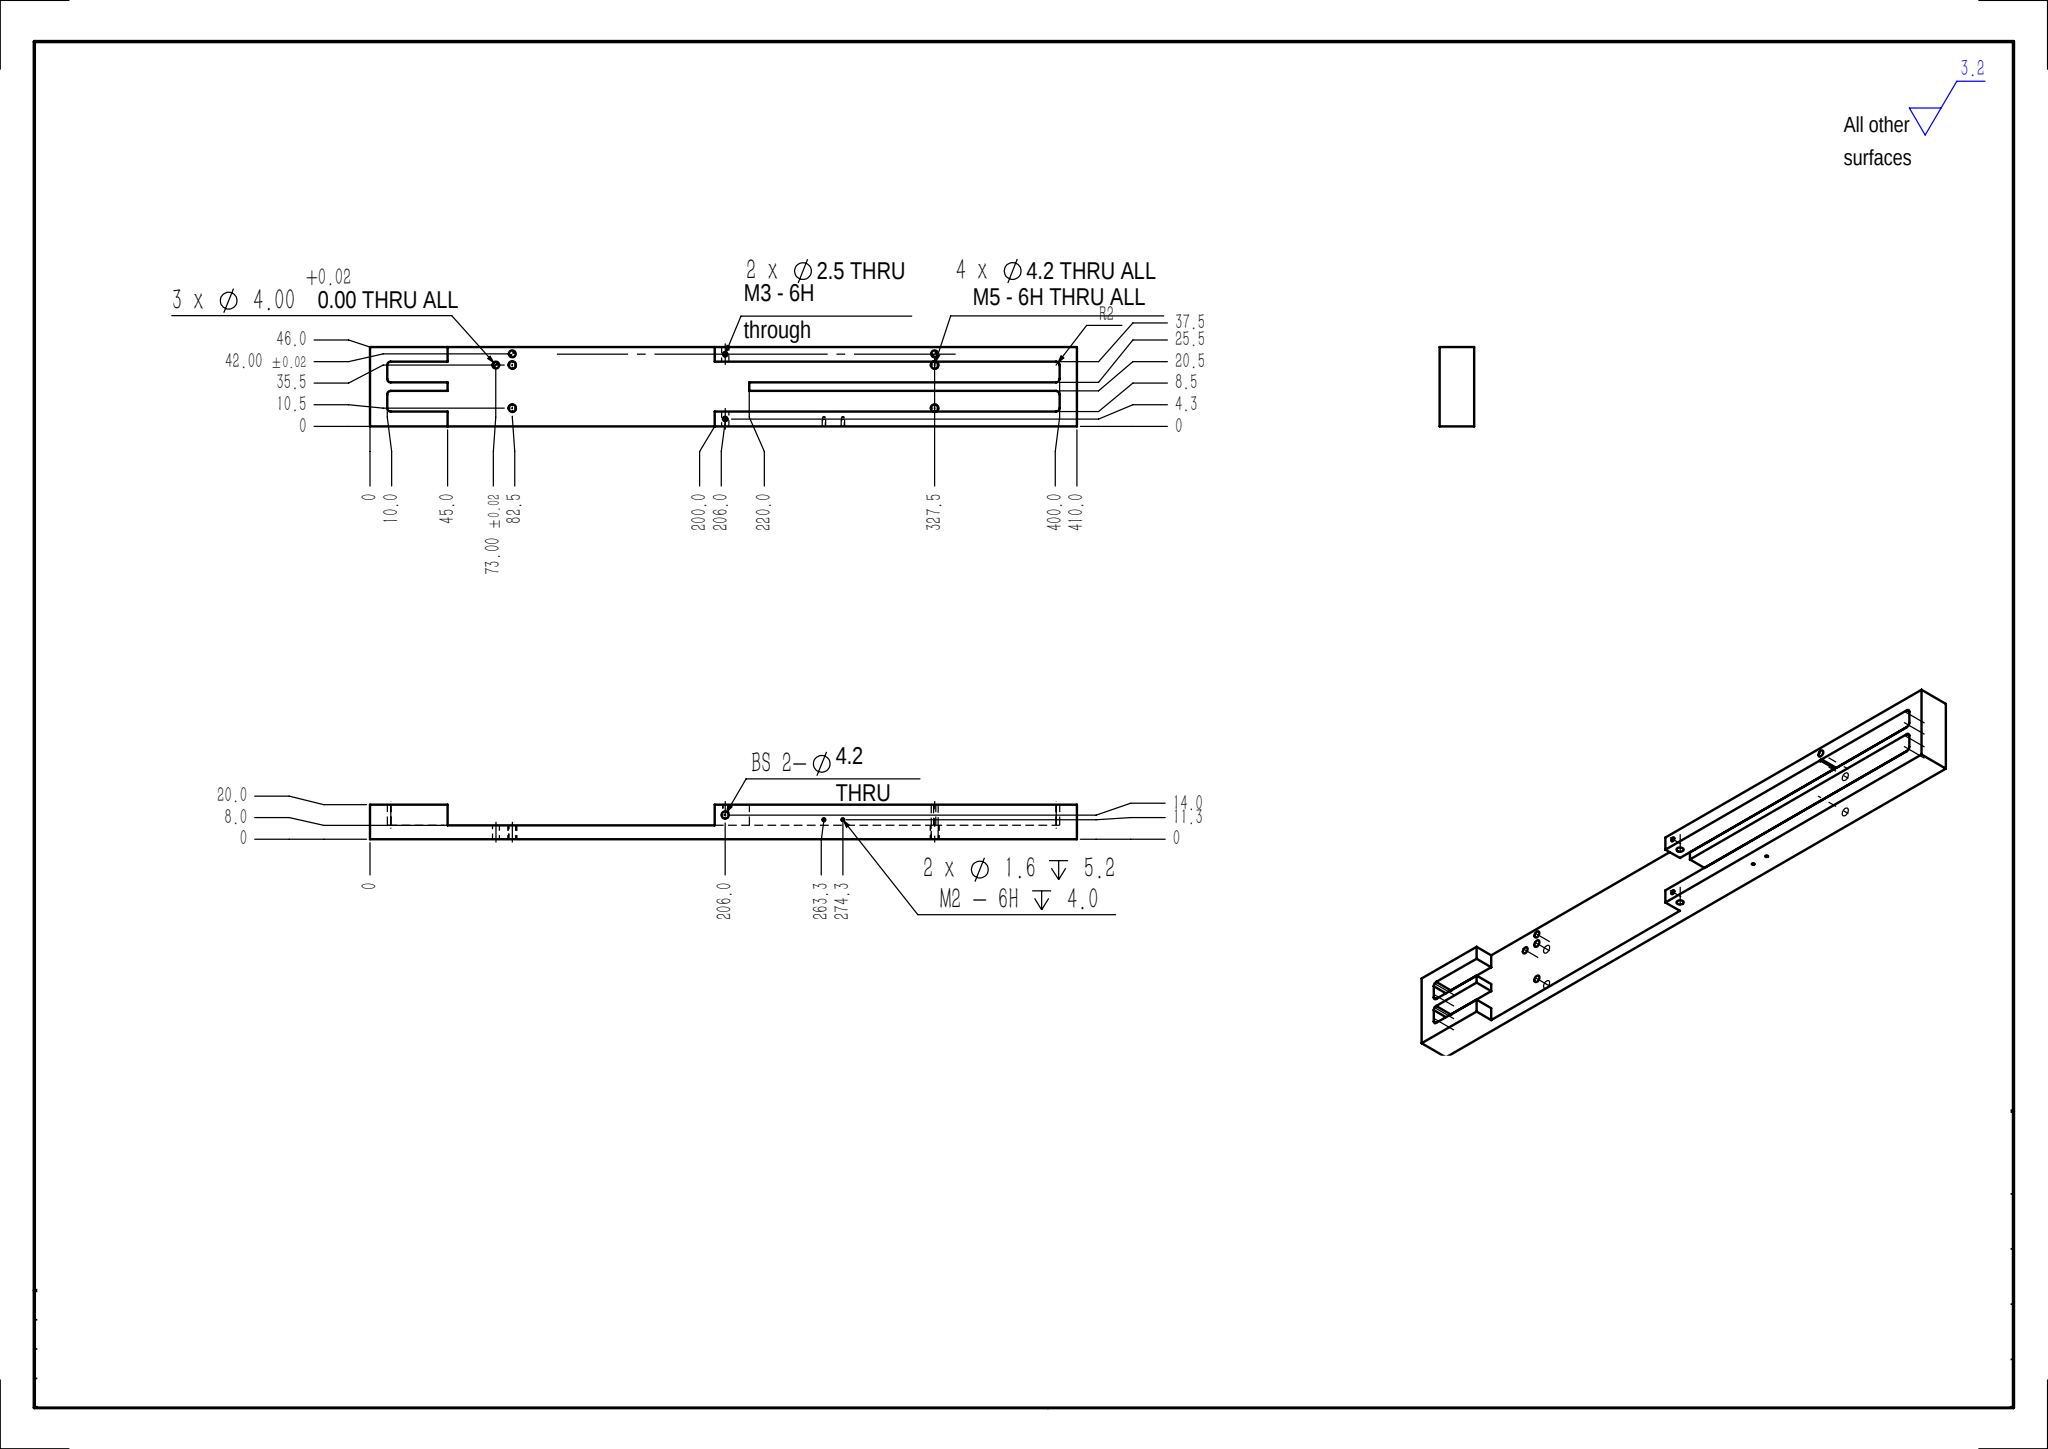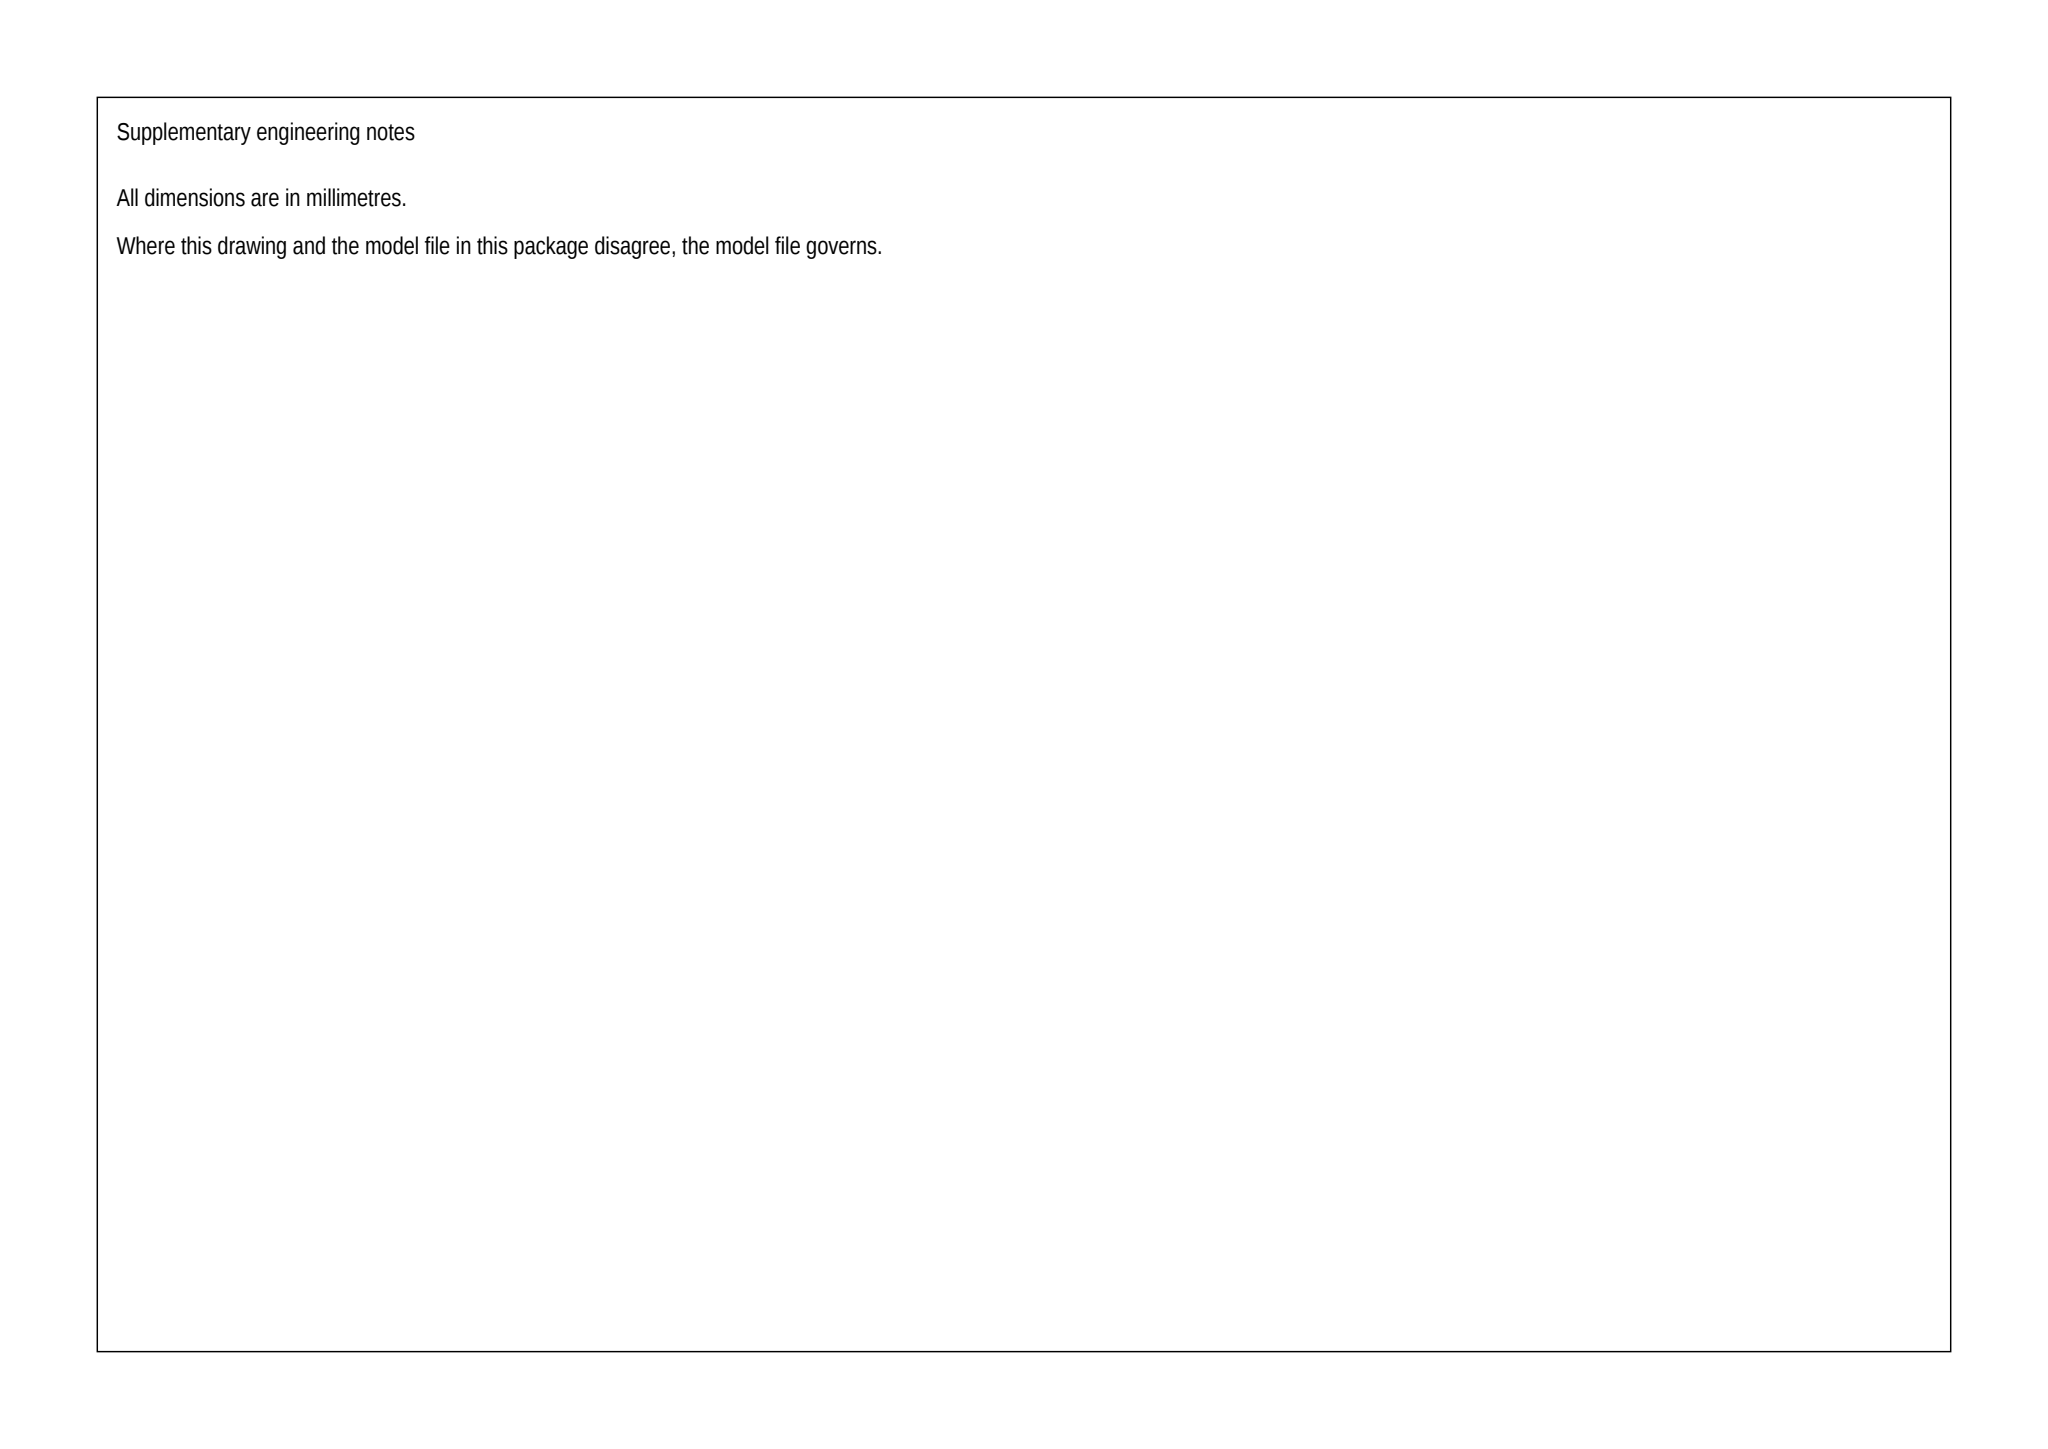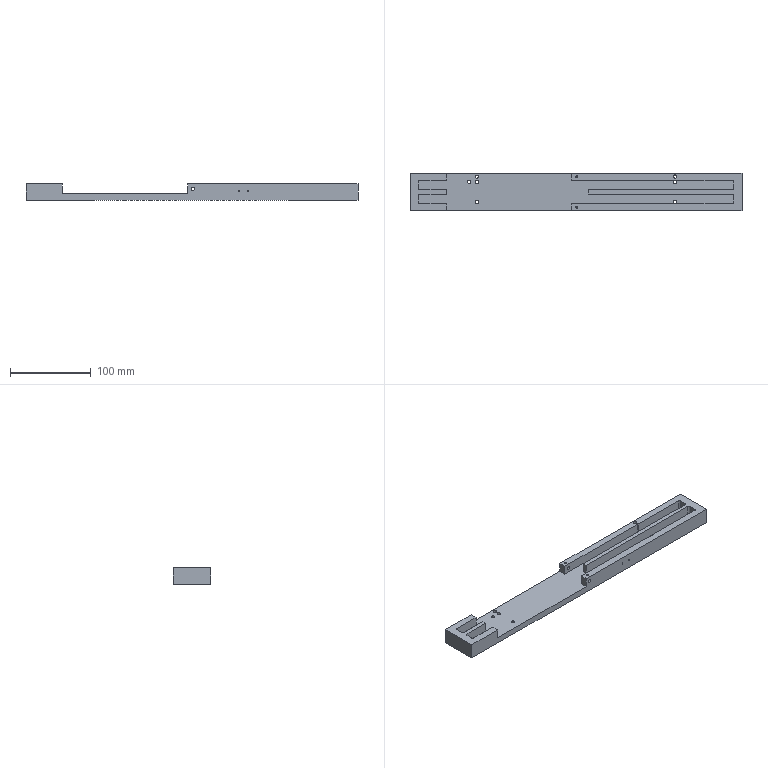Part | SolidWorks | mm | 1 solid | 66 faces | box 410 x 46 x 20 mm | volume 221648 mm3 | cylinder 34 | plane 28 | cone 4 | commonest cylinder face diameters 4 x14 4.2 x12 1.6 x4 2.5 x4
build123d program:
from build123d import *

# Parameters (mm, degrees)
SKETCH1_W                 = 410
SKETCH1_H                 = 46
BOSS_EXTRUDE1_DEPTH       = 10
CUT_EXTRUDE1_START        = -12
CUT_EXTRUDE1_DEPTH        = 12
SKETCH3_W                 = 155
SKETCH3_H                 = 46
CUT_EXTRUDE2_DEPTH        = 12
SKETCH4_W                 = 20
SKETCH4_H                 = 5
CUT_EXTRUDE3_DEPTH        = 12
SKETCH5_R                 = 2.1
CUT_EXTRUDE4_DEPTH        = 211.335
M3_TAPPED_HOLE1_REACH     = 209.253
M3_TAPPED_HOLE1_BORE_R    = 1.25
M5_TAPPED_HOLE1_D         = 4.2
SIZE_MM_DOWEL_PIN_HOLE1_D = 4
M2_TAPPED_HOLE1_D         = 1.6
M2_TAPPED_HOLE1_DEPTH     = 5.2
M2_TAPPED_HOLE1_TIP       = 0.4807


with BuildPart() as part:
    # Sketch1 → Boss-Extrude1 (new, symmetric)
    with BuildSketch(Plane.XY):
        Rectangle(SKETCH1_W, SKETCH1_H)
    extrude(amount=BOSS_EXTRUDE1_DEPTH, both=True)

    # Sketch2 → Cut-Extrude1 (cut)
    with BuildSketch(Plane.XY.offset(10).offset(CUT_EXTRUDE1_START)):
        with BuildLine():
            Line((-193, 14.5), (193, 14.5))
            ThreePointArc((193, 14.5), (194.414, 13.914), (195, 12.5))
            Line((195, 12.5), (195, 4.5))
            ThreePointArc((195, 4.5), (194.414, 3.086), (193, 2.5))
            Line((193, 2.5), (-193, 2.5))
            ThreePointArc((-193, 2.5), (-194.414, 3.086), (-195, 4.5))
            Line((-195, 4.5), (-195, 12.5))
            ThreePointArc((-195, 12.5), (-194.414, 13.914), (-193, 14.5))
        make_face()
        with BuildLine():
            Line((195, -12.5), (195, -4.5))
            ThreePointArc((195, -4.5), (194.414, -3.086), (193, -2.5))
            Line((193, -2.5), (-193, -2.5))
            ThreePointArc((-193, -2.5), (-194.414, -3.086), (-195, -4.5))
            Line((-195, -4.5), (-195, -12.5))
            ThreePointArc((-195, -12.5), (-194.414, -13.914), (-193, -14.5))
            Line((-193, -14.5), (193, -14.5))
            ThreePointArc((193, -14.5), (194.414, -13.914), (195, -12.5))
        make_face()
    extrude(amount=CUT_EXTRUDE1_DEPTH, mode=Mode.SUBTRACT)

    # Sketch3 → Cut-Extrude2 (cut)
    with BuildSketch(Plane.XY.offset(10)):
        with Locations((-82.5, 0)):
            Rectangle(SKETCH3_W, SKETCH3_H)
    extrude(amount=-CUT_EXTRUDE2_DEPTH, mode=Mode.SUBTRACT)

    # Sketch4 → Cut-Extrude3 (cut)
    with BuildSketch(Plane.XY.offset(10)):
        with Locations((5, 0)):
            Rectangle(SKETCH4_W, SKETCH4_H)
    extrude(amount=-CUT_EXTRUDE3_DEPTH, mode=Mode.SUBTRACT)

    # Sketch5 → Cut-Extrude4 (cut, through all)
    with BuildSketch(Plane(origin=(0, -23, 0), x_dir=(-1, 0, 0), z_dir=(0, -1, 0))):
        with Locations(Location((-1, -4, 0), (0, 0, 90))):
            Circle(SKETCH5_R)
    extrude(amount=-CUT_EXTRUDE4_DEPTH, mode=Mode.SUBTRACT)

    # M3 Tapped Hole1 bore → M3 Tapped Hole1 (cut, up to next)
    with BuildSketch(Plane.XY.offset(10), mode=Mode.PRIVATE) as m3_tapped_hole1_sk1:
        with Locations((1, 18.75)):
            Circle(M3_TAPPED_HOLE1_BORE_R)
    m3_tapped_hole1_tool1 = extrude(m3_tapped_hole1_sk1.sketch, amount=-M3_TAPPED_HOLE1_REACH, mode=Mode.PRIVATE) & part.part
    # M3 Tapped Hole1 bore → M3 Tapped Hole1 (cut, up to next)
    with BuildSketch(Plane.XY.offset(10), mode=Mode.PRIVATE) as m3_tapped_hole1_sk2:
        with Locations((1, -18.75)):
            Circle(M3_TAPPED_HOLE1_BORE_R)
    m3_tapped_hole1_tool2 = extrude(m3_tapped_hole1_sk2.sketch, amount=-M3_TAPPED_HOLE1_REACH, mode=Mode.PRIVATE) & part.part
    add(m3_tapped_hole1_tool1.solids().sort_by_distance((1, 18.75, 10))[0], mode=Mode.SUBTRACT)
    add(m3_tapped_hole1_tool2.solids().sort_by_distance((1, -18.75, 10))[0], mode=Mode.SUBTRACT)

    # M5 Tapped Hole1 (through all)
    with Locations(Plane(origin=(0, 0, -10), x_dir=(-1, 0, 0), z_dir=(0, 0, -1))):
        with Locations((122.5, 12.5), (122.5, -12.5), (-122.5, 12.5), (-122.5, -12.5)):
            Hole(M5_TAPPED_HOLE1_D / 2)

    # Size mm Dowel Pin Hole1 (through all)
    with Locations(Plane(origin=(0, 0, -10), x_dir=(-1, 0, 0), z_dir=(0, 0, -1))):
        with Locations((122.5, 19), (132, 12.5), (-122.5, 19)):
            Hole(SIZE_MM_DOWEL_PIN_HOLE1_D / 2)

    # M2 Tapped Hole1
    with Locations(Plane(origin=(0, -23, 0), x_dir=(-1, 0, 0), z_dir=(0, -1, 0))):
        with Locations((-58.25, -1.25), (-69.25, -1.25)):
            Hole(M2_TAPPED_HOLE1_D / 2, depth=M2_TAPPED_HOLE1_DEPTH)
            with Locations((0, 0, -(M2_TAPPED_HOLE1_DEPTH + M2_TAPPED_HOLE1_TIP / 2))):  # 118° drill point
                Cone(0, M2_TAPPED_HOLE1_D / 2, M2_TAPPED_HOLE1_TIP, mode=Mode.SUBTRACT)


solid = part.part